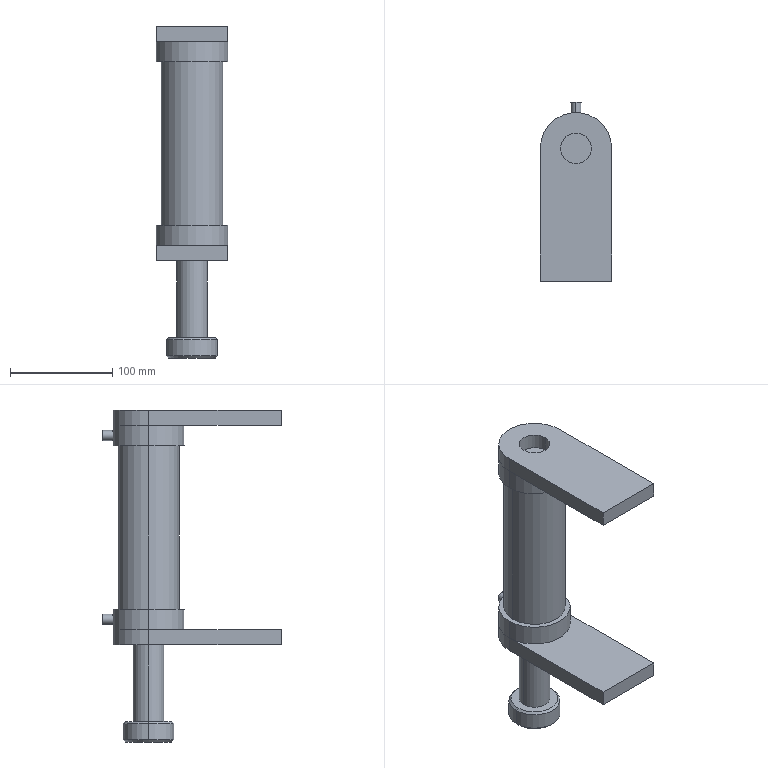Component | SolidWorks | HydraulicCylinderA-1 | 5 solids | 54 faces | box 70 x 175 x 325 mm | volume 1017163 mm3 | cylinder 28 | plane 22 | cone 4 | commonest cylinder face diameters 10 x8 30 x6 70 x6 6 x4 50 x2 60 x2 | material 45
build123d program:
from build123d import *

# Parameters (mm, degrees)
SKETCH2_2_R           = 25
BOSS_EXTRUDE1_DEPTH   = 20
CHAMFER1_SIZE         = 2
SKETCH3_R             = 15
BOSS_EXTRUDE2_DEPTH   = 15
SKETCH2_R             = 5
CUT_EXTRUDE2_DEPTH    = 40
SKETCH4_R             = 5
SKETCH4_R_2           = 3
BOSS_EXTRUDE3_DEPTH   = 45
BOSS_EXTRUDE3_2_DEPTH = 45


with BuildPart() as part:
    # Sketch1 → Revolve1 (revolve)
    with BuildSketch(Plane.XY, mode=Mode.PRIVATE) as revolve1_sk:
        Polygon((0, 0), (0, 15), (90, 15), (90, 35), (110, 35), (110, 30), (270, 30), (270, 35), (290, 35), (290, 0), align=None)
    revolve(revolve1_sk.sketch.rotate(Axis((0, 0, 0), (1, 0, 0)), 180), axis=Axis((0, 0, 0), (1, 0, 0)))

    # Sketch2_2 → Boss-Extrude1 (add)
    with BuildSketch(Plane.ZY):
        with Locations(Location((0, 0, 0), (0, 0, 270))):
            Circle(SKETCH2_2_R)
    extrude(amount=BOSS_EXTRUDE1_DEPTH)

    # Chamfer1
    chamfer1_edges = [part.edges().sort_by_distance(p)[0] for p in [
        (0, 25, 0),
        (-20, 25, 0),
    ]]
    chamfer(chamfer1_edges, length=CHAMFER1_SIZE)

    # Sketch2 → Cut-Extrude2 (cut)
    with BuildSketch(Plane.XY):
        with Locations(Location((100, 0, 0), (0, 0, 180))):
            Circle(SKETCH2_R)
        with Locations(Location((280, 0, 0), (0, 0, 180))):
            Circle(SKETCH2_R)
    extrude(amount=CUT_EXTRUDE2_DEPTH, mode=Mode.SUBTRACT)


with BuildPart() as body_2:
    # Sketch3 → Boss-Extrude2 (new body)
    with BuildSketch(Plane.ZY.offset(-90)):
        with BuildLine():
            Line((0, 35), (-130, 35))
            Line((-130, 35), (-130, -35))
            Line((-130, -35), (0, -35))
            ThreePointArc((0, -35), (35, 0), (0, 35))
        make_face()
        with Locations(Location((0, 0, 0), (0, 0, 270))):
            Circle(SKETCH3_R, mode=Mode.SUBTRACT)
    extrude(amount=BOSS_EXTRUDE2_DEPTH)


with BuildPart() as body_3:
    # Mirror1: mirrored copy
    add(body_2.part.mirror(Plane.ZY.offset(-190)))


with BuildPart() as body_4:
    # Sketch4 → Boss-Extrude3 (new body)
    with BuildSketch(Plane.XY):
        with Locations(Location((100, 0, 0), (0, 0, 180))):
            Circle(SKETCH4_R)
        with Locations(Location((100, 0, 0), (0, 0, 180))):
            Circle(SKETCH4_R_2, mode=Mode.SUBTRACT)
    extrude(amount=BOSS_EXTRUDE3_DEPTH)


with BuildPart() as body_5:
    # Sketch4 → Boss-Extrude3 2 (new body)
    with BuildSketch(Plane.XY):
        with Locations(Location((280, 0, 0), (0, 0, 180))):
            Circle(SKETCH4_R)
        with Locations(Location((280, 0, 0), (0, 0, 180))):
            Circle(SKETCH4_R_2, mode=Mode.SUBTRACT)
    extrude(amount=BOSS_EXTRUDE3_2_DEPTH)


solid = Compound([part.part, body_2.part, body_3.part, body_4.part, body_5.part])

# Placed as in the assembly
solid = solid.moved(Location((-135.812, 248.429, 950), (-90, 0, -90)))